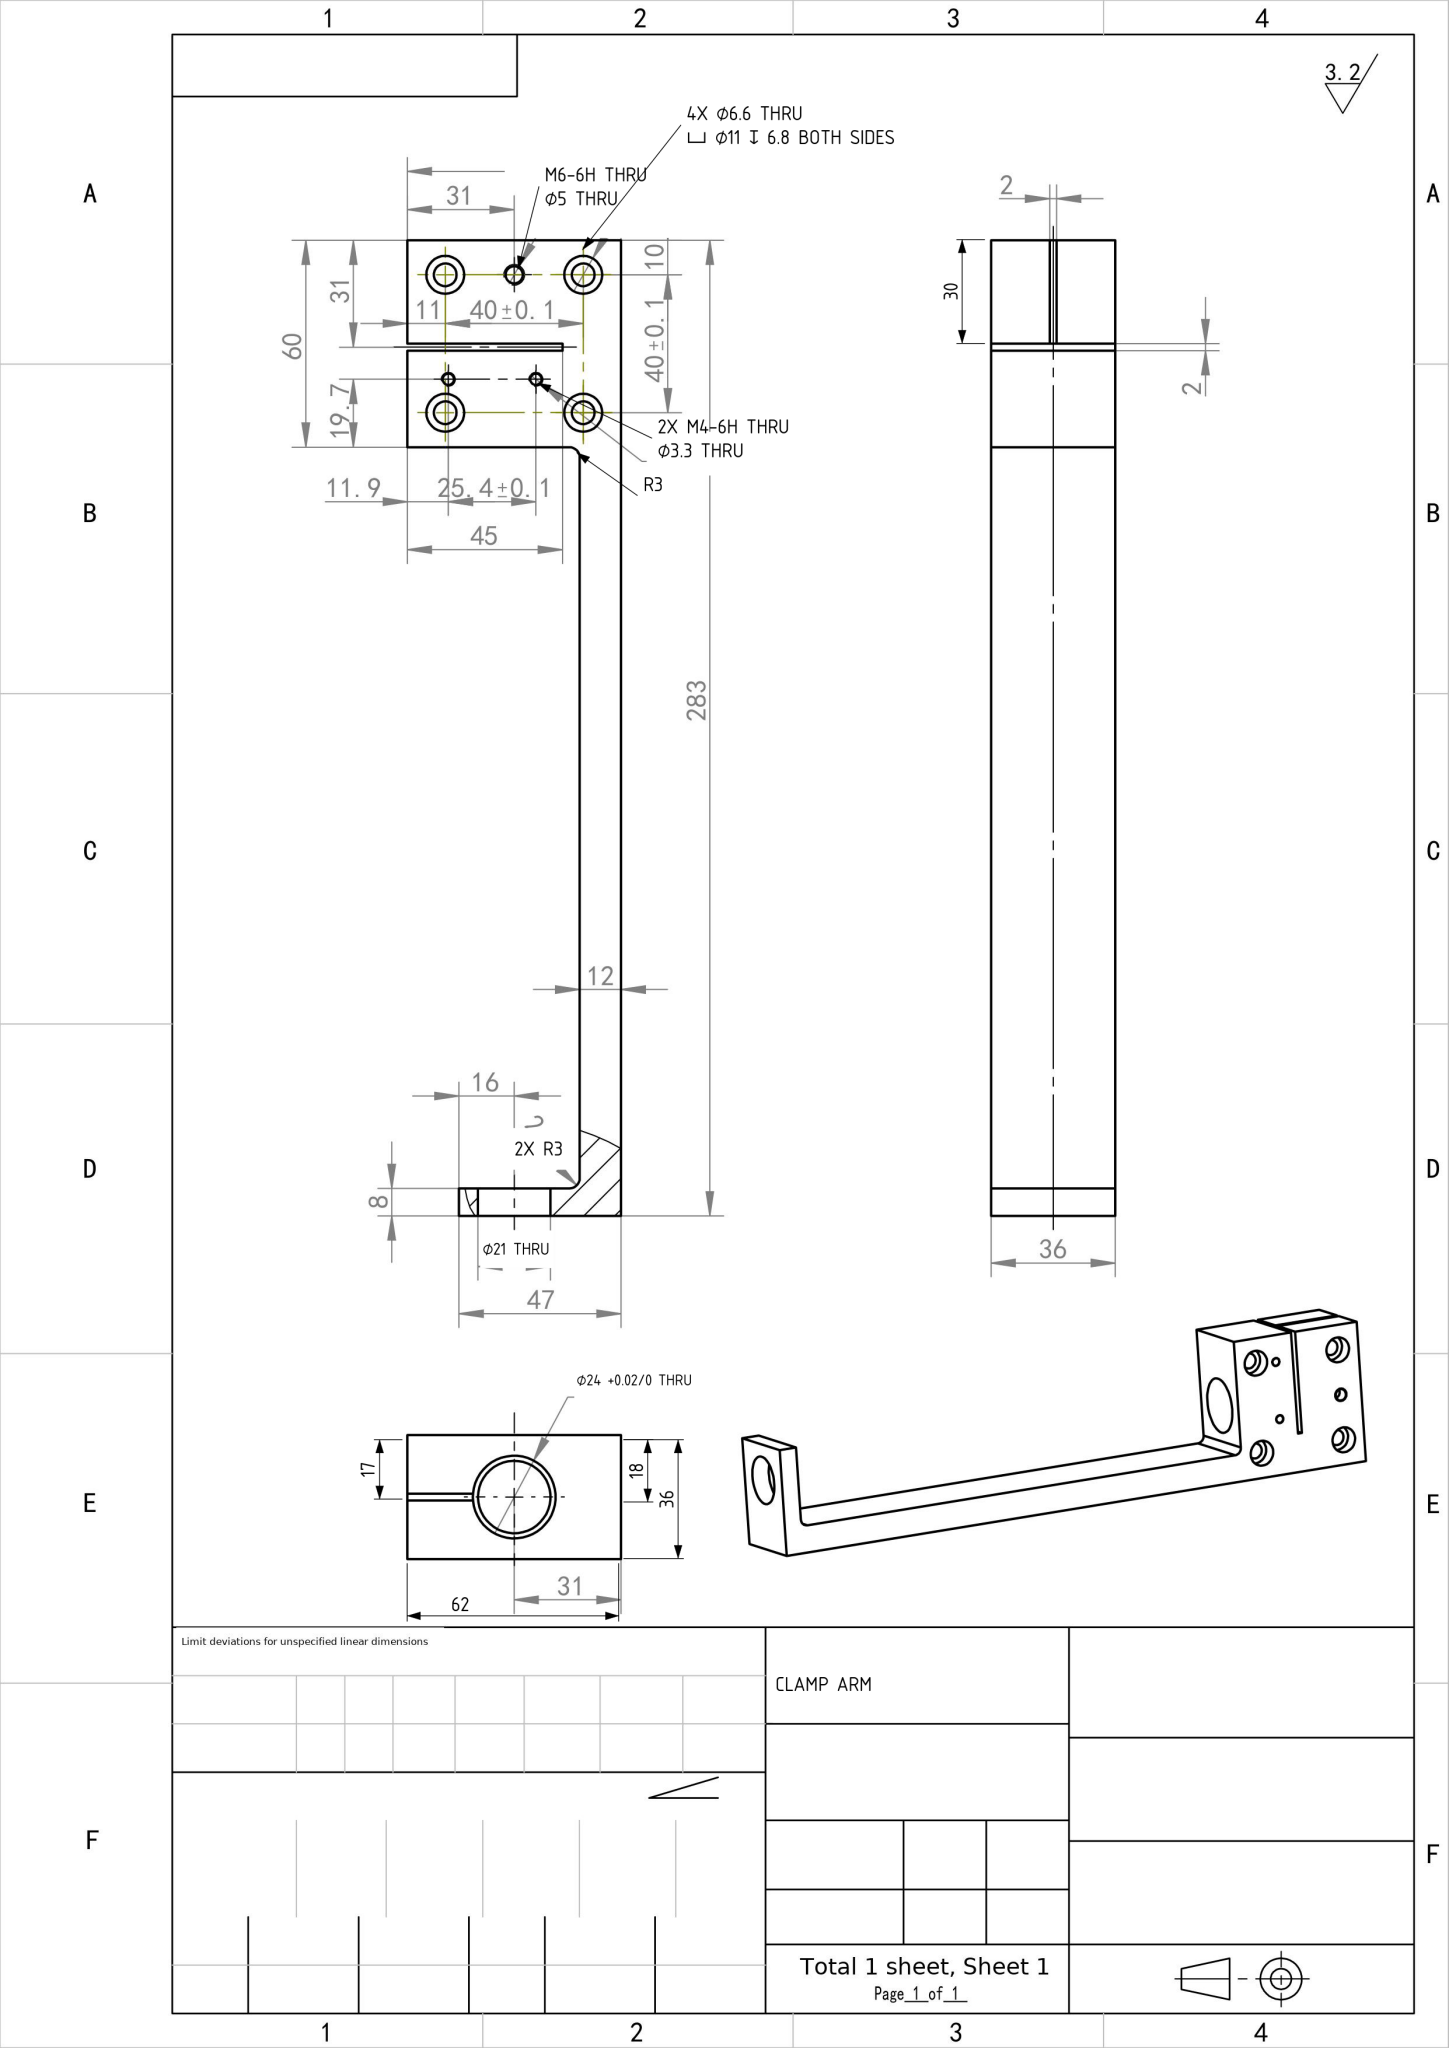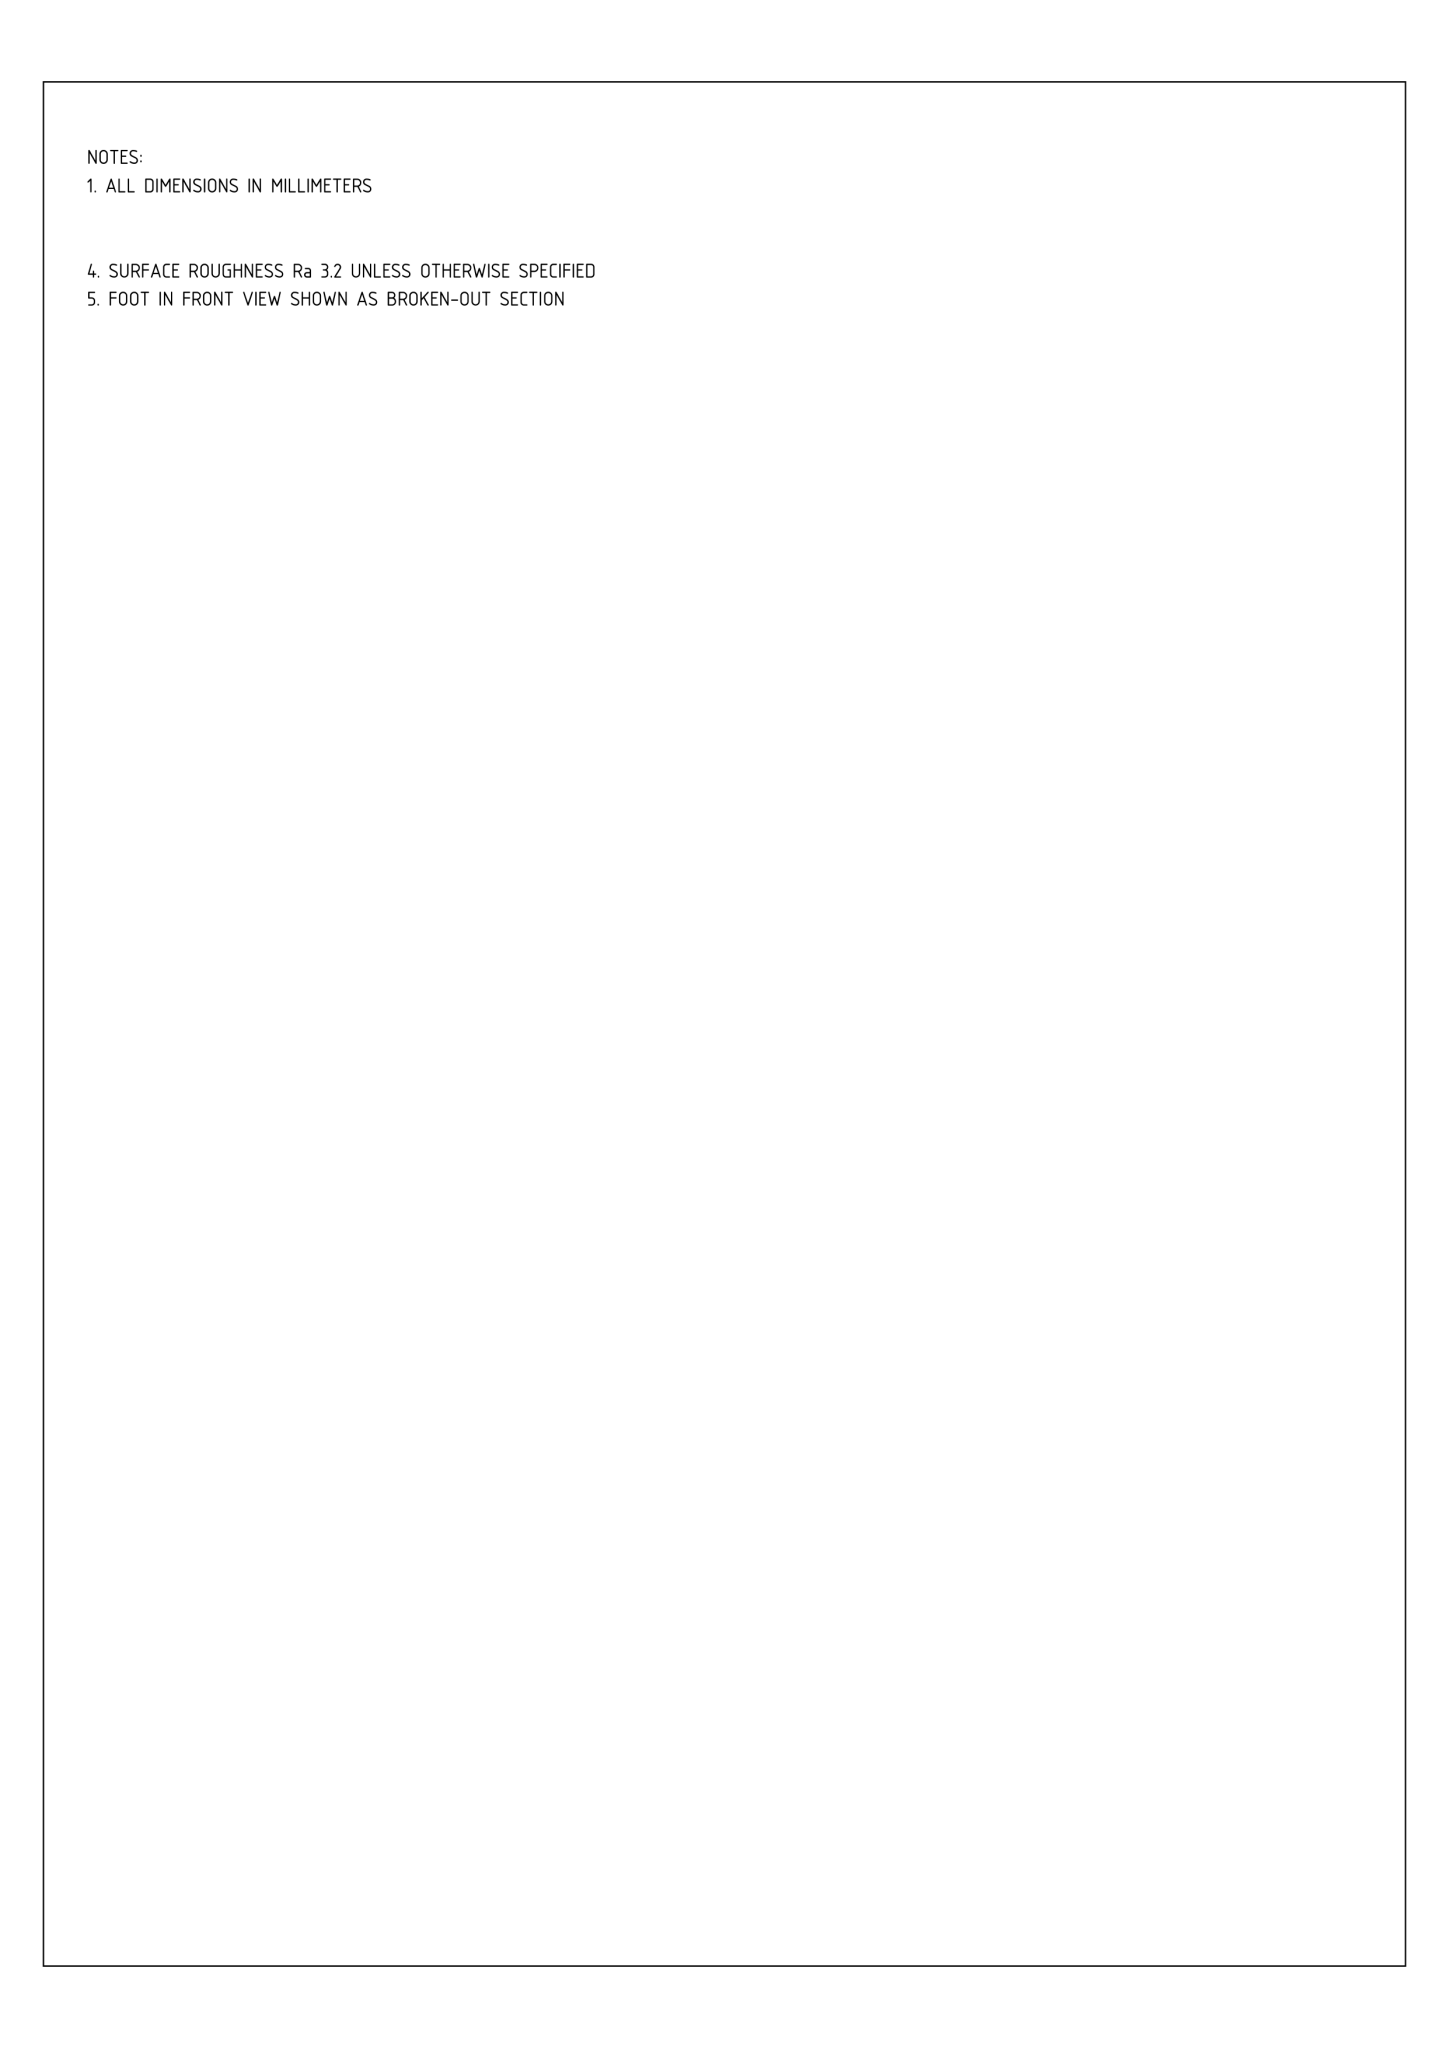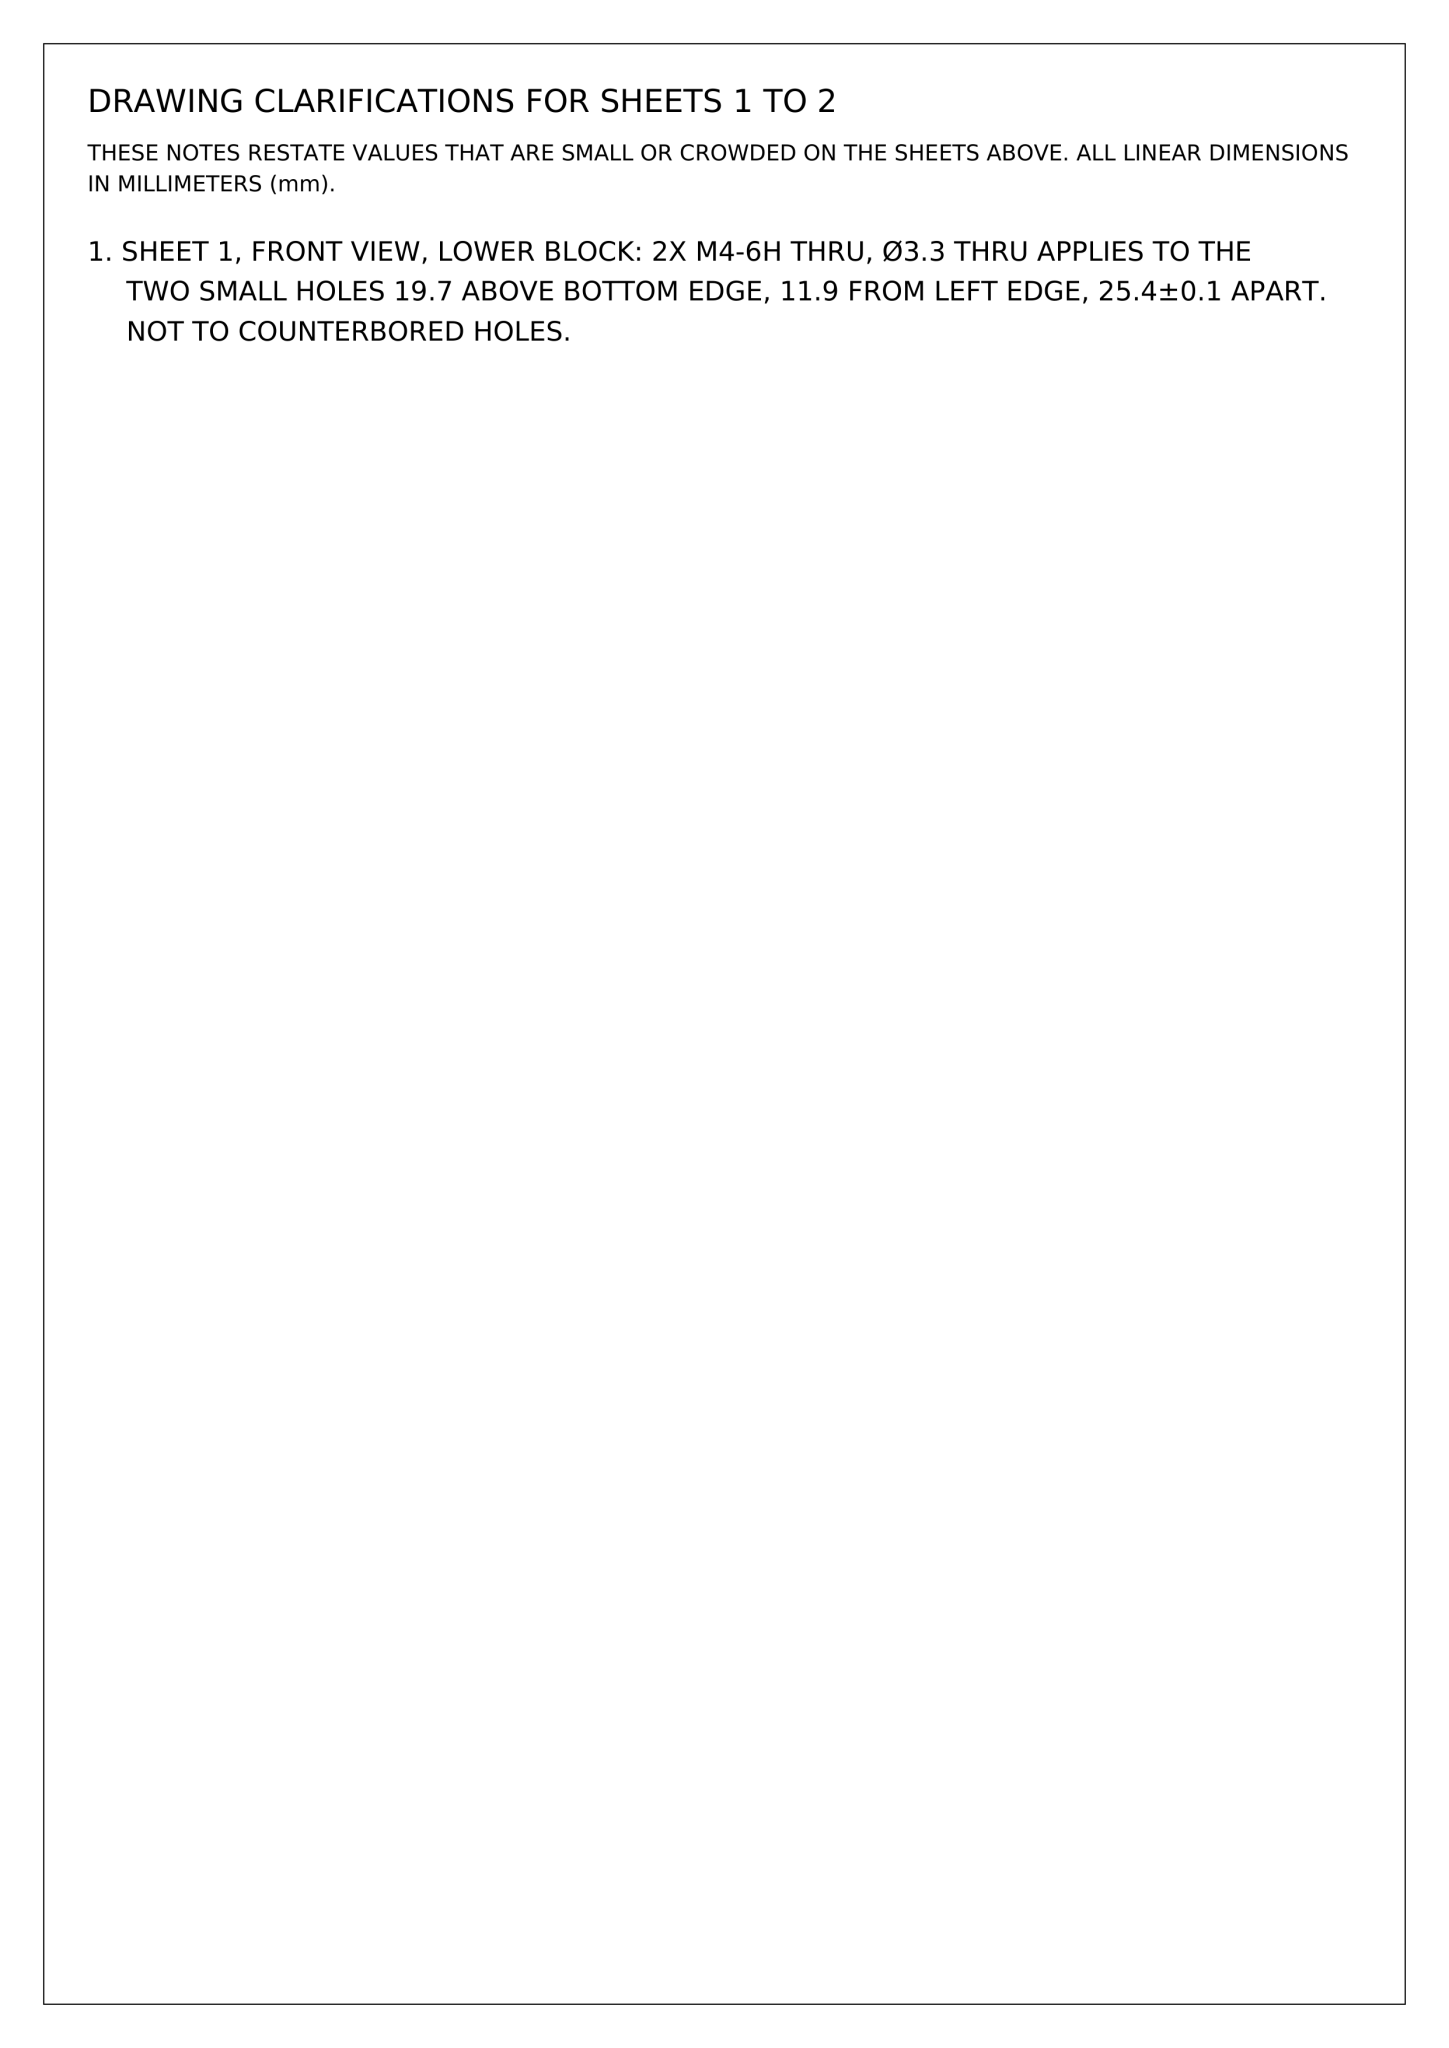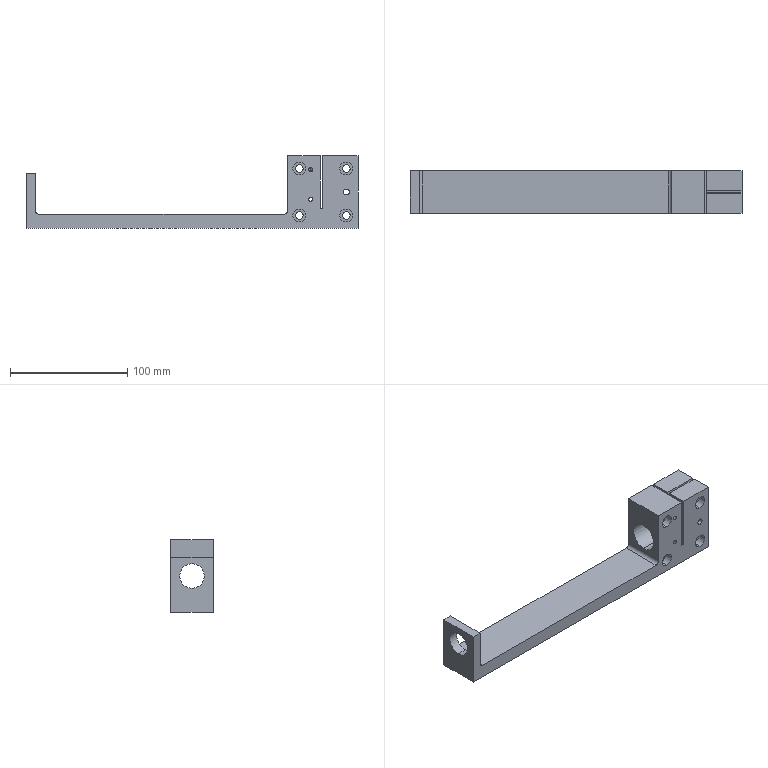Part | NX | mm | 1 solid | 75 faces | box 283 x 36 x 62 mm | volume 198343 mm3 | cylinder 46 | plane 25 | cone 4 | commonest cylinder face diameters 11 x16 6.6 x10 3.3 x8 5 x4 24 x4 21 x2 6 x2